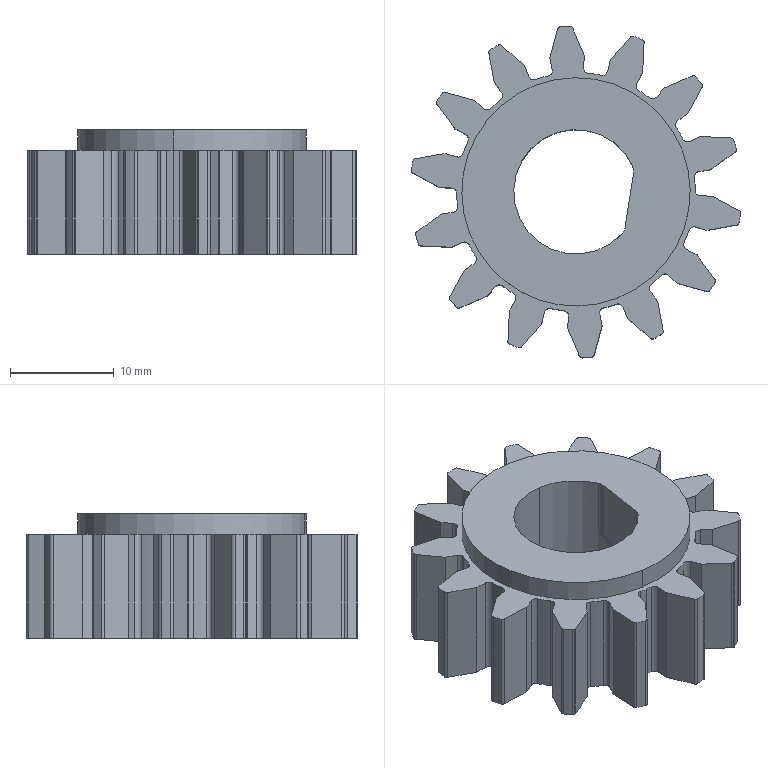Component | SolidWorks | DriveDevice-1_SmallGear-1 | 1 solid | 166 faces | volume 5236 mm3 | cylinder 105 | plane 61 | commonest cylinder face diameters 1 x36 0.6 x34 23 x15 32 x14 12 x2 22 x2 2 x2